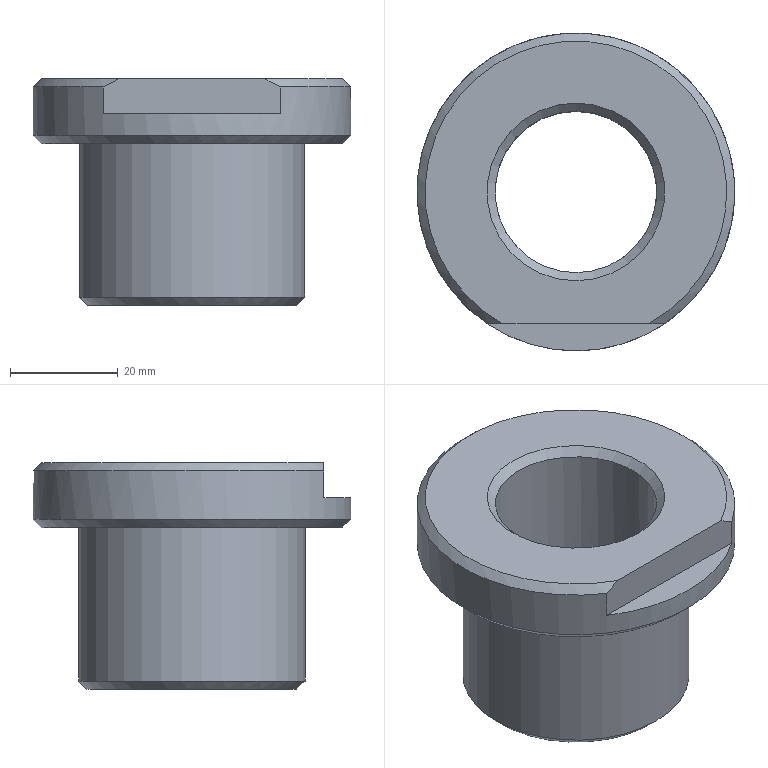Component | NX | BORING_SLEEVE | 1 solid | 13 faces | box 59 x 59 x 42 mm | volume 43221 mm3 | plane 5 | cone 5 | cylinder 3 | commonest cylinder face diameters 42 x1 59 x1 30 x1
STEP:
#1=CARTESIAN_POINT('',(0.,0.,0.));
#2=DIRECTION('',(0.,0.,1.));
#3=DIRECTION('',(1.,0.,0.));
#4=AXIS2_PLACEMENT_3D('',#1,#2,#3);
#5=CARTESIAN_POINT('',(34.,160.533,50.));
#6=VERTEX_POINT('',#5);
#7=CARTESIAN_POINT('',(34.,144.033,50.));
#8=DIRECTION('',(0.,0.,1.));
#9=DIRECTION('',(0.,1.,0.));
#10=AXIS2_PLACEMENT_3D('',#7,#8,#9);
#11=CIRCLE('',#10,16.5);
#12=CARTESIAN_POINT('',(34.,144.033,50.));
#13=DIRECTION('',(0.,0.,-1.));
#14=DIRECTION('',(0.,1.,0.));
#15=AXIS2_PLACEMENT_3D('',#12,#13,#14);
#16=PLANE('',#15);
#17=CARTESIAN_POINT('',(16.5,0.));
#18=CARTESIAN_POINT('',(16.5,-28.579));
#19=CARTESIAN_POINT('',(-8.25,-14.289));
#20=CARTESIAN_POINT('',(-33.,-0.));
#21=CARTESIAN_POINT('',(-8.25,14.289));
#22=CARTESIAN_POINT('',(16.5,28.579));
#23=CARTESIAN_POINT('',(16.5,0.));
#24=(BOUNDED_CURVE()B_SPLINE_CURVE(2,(#17,#18,#19,#20,#21,#22,#23),.UNSPECIFIED.,.T.,.F.)B_SPLINE_CURVE_WITH_KNOTS((1,2,2,2,2,1),(-2.094,0.,2.094,4.189,6.283,8.378),.UNSPECIFIED.)CURVE()GEOMETRIC_REPRESENTATION_ITEM()RATIONAL_B_SPLINE_CURVE((1.,0.5,1.,0.5,1.,0.5,1.))REPRESENTATION_ITEM(''));
#25=(GEOMETRIC_REPRESENTATION_CONTEXT(2)PARAMETRIC_REPRESENTATION_CONTEXT()REPRESENTATION_CONTEXT('',''));
#26=DEFINITIONAL_REPRESENTATION('',(#24),#25);
#27=PCURVE('',#16,#26);
#28=CARTESIAN_POINT('',(34.,144.033,51.5));
#29=DIRECTION('',(0.,0.,-1.));
#30=DIRECTION('',(0.,1.,0.));
#31=AXIS2_PLACEMENT_3D('',#28,#29,#30);
#32=CONICAL_SURFACE('',#31,15.,0.7854);
#33=CARTESIAN_POINT('',(6.283,1.5));
#34=DIRECTION('',(-1.,0.));
#35=VECTOR('',#34,1.);
#36=LINE('',#33,#35);
#37=(GEOMETRIC_REPRESENTATION_CONTEXT(2)PARAMETRIC_REPRESENTATION_CONTEXT()REPRESENTATION_CONTEXT('',''));
#38=DEFINITIONAL_REPRESENTATION('',(#36),#37);
#39=PCURVE('',#32,#38);
#40=SURFACE_CURVE('',#11,(#27,#39),.PCURVE_S1.);
#41=EDGE_CURVE('',#6,#6,#40,.T.);
#42=ORIENTED_EDGE('',*,*,#41,.T.);
#43=EDGE_LOOP('',(#42));
#44=FACE_BOUND('',#43,.T.);
#45=CARTESIAN_POINT('',(34.,163.533,50.));
#46=VERTEX_POINT('',#45);
#47=CARTESIAN_POINT('',(34.,144.033,50.));
#48=DIRECTION('',(0.,0.,-1.));
#49=DIRECTION('',(0.,1.,0.));
#50=AXIS2_PLACEMENT_3D('',#47,#48,#49);
#51=CIRCLE('',#50,19.5);
#52=CARTESIAN_POINT('',(0.,0.));
#53=DIRECTION('',(1.,0.));
#54=AXIS2_PLACEMENT_2D('',#52,#53);
#55=CIRCLE('',#54,19.5);
#56=(GEOMETRIC_REPRESENTATION_CONTEXT(2)PARAMETRIC_REPRESENTATION_CONTEXT()REPRESENTATION_CONTEXT('',''));
#57=DEFINITIONAL_REPRESENTATION('',(#55),#56);
#58=PCURVE('',#16,#57);
#59=CARTESIAN_POINT('',(34.,144.033,51.5));
#60=DIRECTION('',(0.,0.,1.));
#61=DIRECTION('',(0.,-1.,0.));
#62=AXIS2_PLACEMENT_3D('',#59,#60,#61);
#63=CONICAL_SURFACE('',#62,21.,0.7854);
#64=CARTESIAN_POINT('',(9.425,-1.5));
#65=DIRECTION('',(-1.,0.));
#66=VECTOR('',#65,1.);
#67=LINE('',#64,#66);
#68=(GEOMETRIC_REPRESENTATION_CONTEXT(2)PARAMETRIC_REPRESENTATION_CONTEXT()REPRESENTATION_CONTEXT('',''));
#69=DEFINITIONAL_REPRESENTATION('',(#67),#68);
#70=PCURVE('',#63,#69);
#71=SURFACE_CURVE('',#51,(#58,#70),.PCURVE_S1.);
#72=EDGE_CURVE('',#46,#46,#71,.T.);
#73=ORIENTED_EDGE('',*,*,#72,.T.);
#74=EDGE_LOOP('',(#73));
#75=FACE_BOUND('',#74,.T.);
#76=ADVANCED_FACE('',(#44,#75),#16,.T.);
#77=CARTESIAN_POINT('',(34.,165.033,51.5));
#78=VERTEX_POINT('',#77);
#79=CARTESIAN_POINT('',(34.,144.033,51.5));
#80=DIRECTION('',(0.,0.,1.));
#81=DIRECTION('',(0.,1.,0.));
#82=AXIS2_PLACEMENT_3D('',#79,#80,#81);
#83=CIRCLE('',#82,21.);
#84=CARTESIAN_POINT('',(34.,144.033,50.));
#85=DIRECTION('',(0.,0.,1.));
#86=DIRECTION('',(0.,-1.,0.));
#87=AXIS2_PLACEMENT_3D('',#84,#85,#86);
#88=CYLINDRICAL_SURFACE('',#87,21.);
#89=CARTESIAN_POINT('',(3.142,1.5));
#90=DIRECTION('',(1.,0.));
#91=VECTOR('',#90,1.);
#92=LINE('',#89,#91);
#93=(GEOMETRIC_REPRESENTATION_CONTEXT(2)PARAMETRIC_REPRESENTATION_CONTEXT()REPRESENTATION_CONTEXT('',''));
#94=DEFINITIONAL_REPRESENTATION('',(#92),#93);
#95=PCURVE('',#88,#94);
#96=CARTESIAN_POINT('',(3.142,0.));
#97=DIRECTION('',(1.,0.));
#98=VECTOR('',#97,1.);
#99=LINE('',#96,#98);
#100=(GEOMETRIC_REPRESENTATION_CONTEXT(2)PARAMETRIC_REPRESENTATION_CONTEXT()REPRESENTATION_CONTEXT('',''));
#101=DEFINITIONAL_REPRESENTATION('',(#99),#100);
#102=PCURVE('',#63,#101);
#103=SURFACE_CURVE('',#83,(#95,#102),.PCURVE_S1.);
#104=EDGE_CURVE('',#78,#78,#103,.T.);
#105=ORIENTED_EDGE('',*,*,#104,.T.);
#106=CARTESIAN_POINT('',(34.,165.033,80.));
#107=VERTEX_POINT('',#106);
#108=CARTESIAN_POINT('',(34.,165.033,51.5));
#109=CARTESIAN_POINT('',(34.,165.033,80.));
#110=B_SPLINE_CURVE_WITH_KNOTS('',1,(#108,#109),.UNSPECIFIED.,.F.,.F.,(2,2),(1.5,30.),.PIECEWISE_BEZIER_KNOTS.);
#111=CARTESIAN_POINT('',(9.425,0.));
#112=DIRECTION('',(0.,1.));
#113=VECTOR('',#112,1.);
#114=LINE('',#111,#113);
#115=(GEOMETRIC_REPRESENTATION_CONTEXT(2)PARAMETRIC_REPRESENTATION_CONTEXT()REPRESENTATION_CONTEXT('',''));
#116=DEFINITIONAL_REPRESENTATION('',(#114),#115);
#117=PCURVE('',#88,#116);
#118=CARTESIAN_POINT('',(3.142,0.));
#119=DIRECTION('',(0.,1.));
#120=VECTOR('',#119,1.);
#121=LINE('',#118,#120);
#122=(GEOMETRIC_REPRESENTATION_CONTEXT(2)PARAMETRIC_REPRESENTATION_CONTEXT()REPRESENTATION_CONTEXT('',''));
#123=DEFINITIONAL_REPRESENTATION('',(#121),#122);
#124=PCURVE('',#88,#123);
#125=SEAM_CURVE('',#110,(#117,#124),.PCURVE_S1.);
#126=EDGE_CURVE('',#78,#107,#125,.T.);
#127=ORIENTED_EDGE('',*,*,#126,.T.);
#128=CARTESIAN_POINT('',(34.,144.033,80.));
#129=DIRECTION('',(0.,0.,1.));
#130=DIRECTION('',(0.,1.,0.));
#131=AXIS2_PLACEMENT_3D('',#128,#129,#130);
#132=CIRCLE('',#131,21.);
#133=CARTESIAN_POINT('',(3.142,30.));
#134=DIRECTION('',(1.,0.));
#135=VECTOR('',#134,1.);
#136=LINE('',#133,#135);
#137=(GEOMETRIC_REPRESENTATION_CONTEXT(2)PARAMETRIC_REPRESENTATION_CONTEXT()REPRESENTATION_CONTEXT('',''));
#138=DEFINITIONAL_REPRESENTATION('',(#136),#137);
#139=PCURVE('',#88,#138);
#140=CARTESIAN_POINT('',(34.,144.033,80.));
#141=DIRECTION('',(0.,0.,-1.));
#142=DIRECTION('',(0.,1.,0.));
#143=AXIS2_PLACEMENT_3D('',#140,#141,#142);
#144=PLANE('',#143);
#145=CARTESIAN_POINT('',(21.,0.));
#146=CARTESIAN_POINT('',(21.,-36.373));
#147=CARTESIAN_POINT('',(-10.5,-18.187));
#148=CARTESIAN_POINT('',(-42.,-0.));
#149=CARTESIAN_POINT('',(-10.5,18.187));
#150=CARTESIAN_POINT('',(21.,36.373));
#151=CARTESIAN_POINT('',(21.,0.));
#152=(BOUNDED_CURVE()B_SPLINE_CURVE(2,(#145,#146,#147,#148,#149,#150,#151),.UNSPECIFIED.,.T.,.F.)B_SPLINE_CURVE_WITH_KNOTS((1,2,2,2,2,1),(-2.094,0.,2.094,4.189,6.283,8.378),.UNSPECIFIED.)CURVE()GEOMETRIC_REPRESENTATION_ITEM()RATIONAL_B_SPLINE_CURVE((1.,0.5,1.,0.5,1.,0.5,1.))REPRESENTATION_ITEM(''));
#153=(GEOMETRIC_REPRESENTATION_CONTEXT(2)PARAMETRIC_REPRESENTATION_CONTEXT()REPRESENTATION_CONTEXT('',''));
#154=DEFINITIONAL_REPRESENTATION('',(#152),#153);
#155=PCURVE('',#144,#154);
#156=SURFACE_CURVE('',#132,(#139,#155),.PCURVE_S1.);
#157=EDGE_CURVE('',#107,#107,#156,.T.);
#158=ORIENTED_EDGE('',*,*,#157,.F.);
#159=ORIENTED_EDGE('',*,*,#126,.F.);
#160=EDGE_LOOP('',(#105,#127,#158,#159));
#161=FACE_BOUND('',#160,.T.);
#162=ADVANCED_FACE('',(#161),#88,.T.);
#163=CARTESIAN_POINT('',(34.,127.533,92.));
#164=VERTEX_POINT('',#163);
#165=CARTESIAN_POINT('',(34.,144.033,92.));
#166=DIRECTION('',(0.,0.,-1.));
#167=DIRECTION('',(0.,-1.,0.));
#168=AXIS2_PLACEMENT_3D('',#165,#166,#167);
#169=CIRCLE('',#168,16.5);
#170=CARTESIAN_POINT('',(34.,144.033,92.));
#171=DIRECTION('',(0.,0.,1.));
#172=DIRECTION('',(0.,-1.,0.));
#173=AXIS2_PLACEMENT_3D('',#170,#171,#172);
#174=PLANE('',#173);
#175=CARTESIAN_POINT('',(16.5,0.));
#176=CARTESIAN_POINT('',(16.5,-28.579));
#177=CARTESIAN_POINT('',(-8.25,-14.289));
#178=CARTESIAN_POINT('',(-33.,-0.));
#179=CARTESIAN_POINT('',(-8.25,14.289));
#180=CARTESIAN_POINT('',(16.5,28.579));
#181=CARTESIAN_POINT('',(16.5,0.));
#182=(BOUNDED_CURVE()B_SPLINE_CURVE(2,(#175,#176,#177,#178,#179,#180,#181),.UNSPECIFIED.,.T.,.F.)B_SPLINE_CURVE_WITH_KNOTS((1,2,2,2,2,1),(-2.094,0.,2.094,4.189,6.283,8.378),.UNSPECIFIED.)CURVE()GEOMETRIC_REPRESENTATION_ITEM()RATIONAL_B_SPLINE_CURVE((1.,0.5,1.,0.5,1.,0.5,1.))REPRESENTATION_ITEM(''));
#183=(GEOMETRIC_REPRESENTATION_CONTEXT(2)PARAMETRIC_REPRESENTATION_CONTEXT()REPRESENTATION_CONTEXT('',''));
#184=DEFINITIONAL_REPRESENTATION('',(#182),#183);
#185=PCURVE('',#174,#184);
#186=CARTESIAN_POINT('',(34.,144.033,92.));
#187=DIRECTION('',(0.,0.,1.));
#188=DIRECTION('',(0.,-1.,0.));
#189=AXIS2_PLACEMENT_3D('',#186,#187,#188);
#190=CONICAL_SURFACE('',#189,16.5,0.7854);
#191=CARTESIAN_POINT('',(6.283,0.));
#192=DIRECTION('',(-1.,0.));
#193=VECTOR('',#192,1.);
#194=LINE('',#191,#193);
#195=(GEOMETRIC_REPRESENTATION_CONTEXT(2)PARAMETRIC_REPRESENTATION_CONTEXT()REPRESENTATION_CONTEXT('',''));
#196=DEFINITIONAL_REPRESENTATION('',(#194),#195);
#197=PCURVE('',#190,#196);
#198=SURFACE_CURVE('',#169,(#185,#197),.PCURVE_S1.);
#199=EDGE_CURVE('',#164,#164,#198,.T.);
#200=ORIENTED_EDGE('',*,*,#199,.T.);
#201=EDGE_LOOP('',(#200));
#202=FACE_BOUND('',#201,.T.);
#203=CARTESIAN_POINT('',(47.555,119.533,92.));
#204=VERTEX_POINT('',#203);
#205=CARTESIAN_POINT('',(20.445,119.533,92.));
#206=VERTEX_POINT('',#205);
#207=CARTESIAN_POINT('',(67.,119.533,92.));
#208=DIRECTION('',(-1.,-0.,0.));
#209=VECTOR('',#208,1.);
#210=LINE('',#207,#209);
#211=CARTESIAN_POINT('',(24.5,33.));
#212=DIRECTION('',(0.,-1.));
#213=VECTOR('',#212,1.);
#214=LINE('',#211,#213);
#215=(GEOMETRIC_REPRESENTATION_CONTEXT(2)PARAMETRIC_REPRESENTATION_CONTEXT()REPRESENTATION_CONTEXT('',''));
#216=DEFINITIONAL_REPRESENTATION('',(#214),#215);
#217=PCURVE('',#174,#216);
#218=CARTESIAN_POINT('',(67.,119.533,85.5));
#219=DIRECTION('',(-0.,1.,0.));
#220=DIRECTION('',(-1.,-0.,0.));
#221=AXIS2_PLACEMENT_3D('',#218,#219,#220);
#222=PLANE('',#221);
#223=CARTESIAN_POINT('',(0.,6.5));
#224=DIRECTION('',(1.,0.));
#225=VECTOR('',#224,1.);
#226=LINE('',#223,#225);
#227=(GEOMETRIC_REPRESENTATION_CONTEXT(2)PARAMETRIC_REPRESENTATION_CONTEXT()REPRESENTATION_CONTEXT('',''));
#228=DEFINITIONAL_REPRESENTATION('',(#226),#227);
#229=PCURVE('',#222,#228);
#230=SURFACE_CURVE('',#210,(#217,#229),.PCURVE_S1.);
#231=EDGE_CURVE('',#204,#206,#230,.T.);
#232=ORIENTED_EDGE('',*,*,#231,.F.);
#233=CARTESIAN_POINT('',(34.,144.033,92.));
#234=DIRECTION('',(0.,0.,1.));
#235=DIRECTION('',(0.,-1.,0.));
#236=AXIS2_PLACEMENT_3D('',#233,#234,#235);
#237=CIRCLE('',#236,28.);
#238=CARTESIAN_POINT('',(0.,0.));
#239=DIRECTION('',(1.,0.));
#240=AXIS2_PLACEMENT_2D('',#238,#239);
#241=CIRCLE('',#240,28.);
#242=(GEOMETRIC_REPRESENTATION_CONTEXT(2)PARAMETRIC_REPRESENTATION_CONTEXT()REPRESENTATION_CONTEXT('',''));
#243=DEFINITIONAL_REPRESENTATION('',(#241),#242);
#244=PCURVE('',#174,#243);
#245=CARTESIAN_POINT('',(34.,144.033,90.5));
#246=DIRECTION('',(0.,0.,-1.));
#247=DIRECTION('',(0.,1.,0.));
#248=AXIS2_PLACEMENT_3D('',#245,#246,#247);
#249=CONICAL_SURFACE('',#248,29.5,0.7854);
#250=CARTESIAN_POINT('',(9.425,-1.5));
#251=DIRECTION('',(-1.,-0.));
#252=VECTOR('',#251,1.);
#253=LINE('',#250,#252);
#254=(GEOMETRIC_REPRESENTATION_CONTEXT(2)PARAMETRIC_REPRESENTATION_CONTEXT()REPRESENTATION_CONTEXT('',''));
#255=DEFINITIONAL_REPRESENTATION('',(#253),#254);
#256=PCURVE('',#249,#255);
#257=SURFACE_CURVE('',#237,(#244,#256),.PCURVE_S1.);
#258=EDGE_CURVE('',#204,#206,#257,.T.);
#259=ORIENTED_EDGE('',*,*,#258,.T.);
#260=EDGE_LOOP('',(#232,#259));
#261=FACE_BOUND('',#260,.T.);
#262=ADVANCED_FACE('',(#202,#261),#174,.T.);
#263=CARTESIAN_POINT('',(34.,172.033,80.));
#264=VERTEX_POINT('',#263);
#265=CARTESIAN_POINT('',(34.,144.033,80.));
#266=DIRECTION('',(0.,0.,-1.));
#267=DIRECTION('',(0.,1.,0.));
#268=AXIS2_PLACEMENT_3D('',#265,#266,#267);
#269=CIRCLE('',#268,28.);
#270=CARTESIAN_POINT('',(0.,0.));
#271=DIRECTION('',(1.,0.));
#272=AXIS2_PLACEMENT_2D('',#270,#271);
#273=CIRCLE('',#272,28.);
#274=(GEOMETRIC_REPRESENTATION_CONTEXT(2)PARAMETRIC_REPRESENTATION_CONTEXT()REPRESENTATION_CONTEXT('',''));
#275=DEFINITIONAL_REPRESENTATION('',(#273),#274);
#276=PCURVE('',#144,#275);
#277=CARTESIAN_POINT('',(34.,144.033,81.5));
#278=DIRECTION('',(0.,0.,1.));
#279=DIRECTION('',(0.,-1.,0.));
#280=AXIS2_PLACEMENT_3D('',#277,#278,#279);
#281=CONICAL_SURFACE('',#280,29.5,0.7854);
#282=CARTESIAN_POINT('',(9.425,-1.5));
#283=DIRECTION('',(-1.,0.));
#284=VECTOR('',#283,1.);
#285=LINE('',#282,#284);
#286=(GEOMETRIC_REPRESENTATION_CONTEXT(2)PARAMETRIC_REPRESENTATION_CONTEXT()REPRESENTATION_CONTEXT('',''));
#287=DEFINITIONAL_REPRESENTATION('',(#285),#286);
#288=PCURVE('',#281,#287);
#289=SURFACE_CURVE('',#269,(#276,#288),.PCURVE_S1.);
#290=EDGE_CURVE('',#264,#264,#289,.T.);
#291=ORIENTED_EDGE('',*,*,#290,.T.);
#292=EDGE_LOOP('',(#291));
#293=FACE_BOUND('',#292,.T.);
#294=ORIENTED_EDGE('',*,*,#157,.T.);
#295=EDGE_LOOP('',(#294));
#296=FACE_BOUND('',#295,.T.);
#297=ADVANCED_FACE('',(#293,#296),#144,.T.);
#298=CARTESIAN_POINT('',(34.,173.533,81.5));
#299=VERTEX_POINT('',#298);
#300=CARTESIAN_POINT('',(17.568,119.533,81.5));
#301=VERTEX_POINT('',#300);
#302=CARTESIAN_POINT('',(34.,144.033,81.5));
#303=DIRECTION('',(0.,0.,1.));
#304=DIRECTION('',(0.,1.,0.));
#305=AXIS2_PLACEMENT_3D('',#302,#303,#304);
#306=CIRCLE('',#305,29.5);
#307=CARTESIAN_POINT('',(34.,144.033,80.));
#308=DIRECTION('',(0.,0.,1.));
#309=DIRECTION('',(0.,-1.,0.));
#310=AXIS2_PLACEMENT_3D('',#307,#308,#309);
#311=CYLINDRICAL_SURFACE('',#310,29.5);
#312=CARTESIAN_POINT('',(9.425,1.5));
#313=DIRECTION('',(1.,0.));
#314=VECTOR('',#313,1.);
#315=LINE('',#312,#314);
#316=(GEOMETRIC_REPRESENTATION_CONTEXT(2)PARAMETRIC_REPRESENTATION_CONTEXT()REPRESENTATION_CONTEXT('',''));
#317=DEFINITIONAL_REPRESENTATION('',(#315),#316);
#318=PCURVE('',#311,#317);
#319=CARTESIAN_POINT('',(3.142,0.));
#320=DIRECTION('',(1.,0.));
#321=VECTOR('',#320,1.);
#322=LINE('',#319,#321);
#323=(GEOMETRIC_REPRESENTATION_CONTEXT(2)PARAMETRIC_REPRESENTATION_CONTEXT()REPRESENTATION_CONTEXT('',''));
#324=DEFINITIONAL_REPRESENTATION('',(#322),#323);
#325=PCURVE('',#281,#324);
#326=SURFACE_CURVE('',#306,(#318,#325),.PCURVE_S1.);
#327=EDGE_CURVE('',#299,#301,#326,.T.);
#328=ORIENTED_EDGE('',*,*,#327,.T.);
#329=CARTESIAN_POINT('',(17.568,119.533,85.5));
#330=VERTEX_POINT('',#329);
#331=CARTESIAN_POINT('',(17.568,119.533,81.5));
#332=CARTESIAN_POINT('',(17.568,119.533,85.5));
#333=B_SPLINE_CURVE_WITH_KNOTS('',1,(#331,#332),.UNSPECIFIED.,.F.,.F.,(2,2),(1.5,5.5),.PIECEWISE_BEZIER_KNOTS.);
#334=CARTESIAN_POINT('',(11.976,0.));
#335=DIRECTION('',(0.,1.));
#336=VECTOR('',#335,1.);
#337=LINE('',#334,#336);
#338=(GEOMETRIC_REPRESENTATION_CONTEXT(2)PARAMETRIC_REPRESENTATION_CONTEXT()REPRESENTATION_CONTEXT('',''));
#339=DEFINITIONAL_REPRESENTATION('',(#337),#338);
#340=PCURVE('',#311,#339);
#341=CARTESIAN_POINT('',(5.692,0.));
#342=DIRECTION('',(0.,1.));
#343=VECTOR('',#342,1.);
#344=LINE('',#341,#343);
#345=(GEOMETRIC_REPRESENTATION_CONTEXT(2)PARAMETRIC_REPRESENTATION_CONTEXT()REPRESENTATION_CONTEXT('',''));
#346=DEFINITIONAL_REPRESENTATION('',(#344),#345);
#347=PCURVE('',#311,#346);
#348=SEAM_CURVE('',#333,(#340,#347),.PCURVE_S1.);
#349=EDGE_CURVE('',#301,#330,#348,.T.);
#350=ORIENTED_EDGE('',*,*,#349,.T.);
#351=CARTESIAN_POINT('',(17.568,119.533,90.5));
#352=VERTEX_POINT('',#351);
#353=CARTESIAN_POINT('',(17.568,119.533,80.));
#354=DIRECTION('',(0.,0.,-1.));
#355=VECTOR('',#354,1.);
#356=LINE('',#353,#355);
#357=CARTESIAN_POINT('',(11.976,0.));
#358=DIRECTION('',(0.,-1.));
#359=VECTOR('',#358,1.);
#360=LINE('',#357,#359);
#361=(GEOMETRIC_REPRESENTATION_CONTEXT(2)PARAMETRIC_REPRESENTATION_CONTEXT()REPRESENTATION_CONTEXT('',''));
#362=DEFINITIONAL_REPRESENTATION('',(#360),#361);
#363=PCURVE('',#311,#362);
#364=CARTESIAN_POINT('',(49.432,-5.5));
#365=DIRECTION('',(0.,-1.));
#366=VECTOR('',#365,1.);
#367=LINE('',#364,#366);
#368=(GEOMETRIC_REPRESENTATION_CONTEXT(2)PARAMETRIC_REPRESENTATION_CONTEXT()REPRESENTATION_CONTEXT('',''));
#369=DEFINITIONAL_REPRESENTATION('',(#367),#368);
#370=PCURVE('',#222,#369);
#371=SURFACE_CURVE('',#356,(#363,#370),.PCURVE_S1.);
#372=EDGE_CURVE('',#352,#330,#371,.T.);
#373=ORIENTED_EDGE('',*,*,#372,.F.);
#374=CARTESIAN_POINT('',(50.432,119.533,90.5));
#375=VERTEX_POINT('',#374);
#376=CARTESIAN_POINT('',(34.,144.033,90.5));
#377=DIRECTION('',(0.,0.,-1.));
#378=DIRECTION('',(0.,-1.,0.));
#379=AXIS2_PLACEMENT_3D('',#376,#377,#378);
#380=CIRCLE('',#379,29.5);
#381=CARTESIAN_POINT('',(12.566,10.5));
#382=DIRECTION('',(-1.,0.));
#383=VECTOR('',#382,1.);
#384=LINE('',#381,#383);
#385=(GEOMETRIC_REPRESENTATION_CONTEXT(2)PARAMETRIC_REPRESENTATION_CONTEXT()REPRESENTATION_CONTEXT('',''));
#386=DEFINITIONAL_REPRESENTATION('',(#384),#385);
#387=PCURVE('',#311,#386);
#388=CARTESIAN_POINT('',(3.142,0.));
#389=DIRECTION('',(1.,-0.));
#390=VECTOR('',#389,1.);
#391=LINE('',#388,#390);
#392=(GEOMETRIC_REPRESENTATION_CONTEXT(2)PARAMETRIC_REPRESENTATION_CONTEXT()REPRESENTATION_CONTEXT('',''));
#393=DEFINITIONAL_REPRESENTATION('',(#391),#392);
#394=PCURVE('',#249,#393);
#395=SURFACE_CURVE('',#380,(#387,#394),.PCURVE_S1.);
#396=EDGE_CURVE('',#352,#375,#395,.T.);
#397=ORIENTED_EDGE('',*,*,#396,.T.);
#398=CARTESIAN_POINT('',(50.432,119.533,85.5));
#399=VERTEX_POINT('',#398);
#400=CARTESIAN_POINT('',(50.432,119.533,80.));
#401=DIRECTION('',(0.,0.,1.));
#402=VECTOR('',#401,1.);
#403=LINE('',#400,#402);
#404=CARTESIAN_POINT('',(6.874,0.));
#405=DIRECTION('',(0.,1.));
#406=VECTOR('',#405,1.);
#407=LINE('',#404,#406);
#408=(GEOMETRIC_REPRESENTATION_CONTEXT(2)PARAMETRIC_REPRESENTATION_CONTEXT()REPRESENTATION_CONTEXT('',''));
#409=DEFINITIONAL_REPRESENTATION('',(#407),#408);
#410=PCURVE('',#311,#409);
#411=CARTESIAN_POINT('',(16.568,-5.5));
#412=DIRECTION('',(0.,1.));
#413=VECTOR('',#412,1.);
#414=LINE('',#411,#413);
#415=(GEOMETRIC_REPRESENTATION_CONTEXT(2)PARAMETRIC_REPRESENTATION_CONTEXT()REPRESENTATION_CONTEXT('',''));
#416=DEFINITIONAL_REPRESENTATION('',(#414),#415);
#417=PCURVE('',#222,#416);
#418=SURFACE_CURVE('',#403,(#410,#417),.PCURVE_S1.);
#419=EDGE_CURVE('',#399,#375,#418,.T.);
#420=ORIENTED_EDGE('',*,*,#419,.F.);
#421=CARTESIAN_POINT('',(34.,144.033,85.5));
#422=DIRECTION('',(0.,0.,-1.));
#423=DIRECTION('',(0.,-1.,0.));
#424=AXIS2_PLACEMENT_3D('',#421,#422,#423);
#425=CIRCLE('',#424,29.5);
#426=CARTESIAN_POINT('',(12.566,5.5));
#427=DIRECTION('',(-1.,0.));
#428=VECTOR('',#427,1.);
#429=LINE('',#426,#428);
#430=(GEOMETRIC_REPRESENTATION_CONTEXT(2)PARAMETRIC_REPRESENTATION_CONTEXT()REPRESENTATION_CONTEXT('',''));
#431=DEFINITIONAL_REPRESENTATION('',(#429),#430);
#432=PCURVE('',#311,#431);
#433=CARTESIAN_POINT('',(34.,144.033,85.5));
#434=DIRECTION('',(0.,0.,1.));
#435=DIRECTION('',(0.,-1.,0.));
#436=AXIS2_PLACEMENT_3D('',#433,#434,#435);
#437=PLANE('',#436);
#438=CARTESIAN_POINT('',(29.5,0.));
#439=CARTESIAN_POINT('',(29.5,-51.095));
#440=CARTESIAN_POINT('',(-14.75,-25.548));
#441=CARTESIAN_POINT('',(-59.,-0.));
#442=CARTESIAN_POINT('',(-14.75,25.548));
#443=CARTESIAN_POINT('',(29.5,51.095));
#444=CARTESIAN_POINT('',(29.5,0.));
#445=(BOUNDED_CURVE()B_SPLINE_CURVE(2,(#438,#439,#440,#441,#442,#443,#444),.UNSPECIFIED.,.T.,.F.)B_SPLINE_CURVE_WITH_KNOTS((1,2,2,2,2,1),(-2.094,0.,2.094,4.189,6.283,8.378),.UNSPECIFIED.)CURVE()GEOMETRIC_REPRESENTATION_ITEM()RATIONAL_B_SPLINE_CURVE((1.,0.5,1.,0.5,1.,0.5,1.))REPRESENTATION_ITEM(''));
#446=(GEOMETRIC_REPRESENTATION_CONTEXT(2)PARAMETRIC_REPRESENTATION_CONTEXT()REPRESENTATION_CONTEXT('',''));
#447=DEFINITIONAL_REPRESENTATION('',(#445),#446);
#448=PCURVE('',#437,#447);
#449=SURFACE_CURVE('',#425,(#432,#448),.PCURVE_S1.);
#450=EDGE_CURVE('',#399,#330,#449,.T.);
#451=ORIENTED_EDGE('',*,*,#450,.T.);
#452=ORIENTED_EDGE('',*,*,#349,.F.);
#453=CARTESIAN_POINT('',(34.,144.033,81.5));
#454=DIRECTION('',(0.,0.,1.));
#455=DIRECTION('',(0.,1.,0.));
#456=AXIS2_PLACEMENT_3D('',#453,#454,#455);
#457=CIRCLE('',#456,29.5);
#458=CARTESIAN_POINT('',(3.142,1.5));
#459=DIRECTION('',(1.,0.));
#460=VECTOR('',#459,1.);
#461=LINE('',#458,#460);
#462=(GEOMETRIC_REPRESENTATION_CONTEXT(2)PARAMETRIC_REPRESENTATION_CONTEXT()REPRESENTATION_CONTEXT('',''));
#463=DEFINITIONAL_REPRESENTATION('',(#461),#462);
#464=PCURVE('',#311,#463);
#465=CARTESIAN_POINT('',(3.142,0.));
#466=DIRECTION('',(1.,0.));
#467=VECTOR('',#466,1.);
#468=LINE('',#465,#467);
#469=(GEOMETRIC_REPRESENTATION_CONTEXT(2)PARAMETRIC_REPRESENTATION_CONTEXT()REPRESENTATION_CONTEXT('',''));
#470=DEFINITIONAL_REPRESENTATION('',(#468),#469);
#471=PCURVE('',#281,#470);
#472=SURFACE_CURVE('',#457,(#464,#471),.PCURVE_S1.);
#473=EDGE_CURVE('',#301,#299,#472,.T.);
#474=ORIENTED_EDGE('',*,*,#473,.T.);
#475=EDGE_LOOP('',(#328,#350,#373,#397,#420,#451,#452,#474));
#476=FACE_BOUND('',#475,.T.);
#477=ADVANCED_FACE('',(#476),#311,.T.);
#478=CARTESIAN_POINT('',(34.,159.033,51.5));
#479=VERTEX_POINT('',#478);
#480=CARTESIAN_POINT('',(34.,144.033,51.5));
#481=DIRECTION('',(0.,0.,-1.));
#482=DIRECTION('',(0.,1.,0.));
#483=AXIS2_PLACEMENT_3D('',#480,#481,#482);
#484=CIRCLE('',#483,15.);
#485=CARTESIAN_POINT('',(34.,144.033,92.));
#486=DIRECTION('',(0.,0.,-1.));
#487=DIRECTION('',(0.,1.,0.));
#488=AXIS2_PLACEMENT_3D('',#485,#486,#487);
#489=CYLINDRICAL_SURFACE('',#488,15.);
#490=CARTESIAN_POINT('',(0.,40.5));
#491=DIRECTION('',(1.,0.));
#492=VECTOR('',#491,1.);
#493=LINE('',#490,#492);
#494=(GEOMETRIC_REPRESENTATION_CONTEXT(2)PARAMETRIC_REPRESENTATION_CONTEXT()REPRESENTATION_CONTEXT('',''));
#495=DEFINITIONAL_REPRESENTATION('',(#493),#494);
#496=PCURVE('',#489,#495);
#497=CARTESIAN_POINT('',(0.,0.));
#498=DIRECTION('',(1.,0.));
#499=VECTOR('',#498,1.);
#500=LINE('',#497,#499);
#501=(GEOMETRIC_REPRESENTATION_CONTEXT(2)PARAMETRIC_REPRESENTATION_CONTEXT()REPRESENTATION_CONTEXT('',''));
#502=DEFINITIONAL_REPRESENTATION('',(#500),#501);
#503=PCURVE('',#32,#502);
#504=SURFACE_CURVE('',#484,(#496,#503),.PCURVE_S1.);
#505=EDGE_CURVE('',#479,#479,#504,.T.);
#506=ORIENTED_EDGE('',*,*,#505,.F.);
#507=CARTESIAN_POINT('',(34.,159.033,90.5));
#508=VERTEX_POINT('',#507);
#509=CARTESIAN_POINT('',(34.,159.033,90.5));
#510=CARTESIAN_POINT('',(34.,159.033,51.5));
#511=B_SPLINE_CURVE_WITH_KNOTS('',1,(#509,#510),.UNSPECIFIED.,.F.,.F.,(2,2),(1.5,40.5),.PIECEWISE_BEZIER_KNOTS.);
#512=CARTESIAN_POINT('',(0.,0.));
#513=DIRECTION('',(0.,1.));
#514=VECTOR('',#513,1.);
#515=LINE('',#512,#514);
#516=(GEOMETRIC_REPRESENTATION_CONTEXT(2)PARAMETRIC_REPRESENTATION_CONTEXT()REPRESENTATION_CONTEXT('',''));
#517=DEFINITIONAL_REPRESENTATION('',(#515),#516);
#518=PCURVE('',#489,#517);
#519=CARTESIAN_POINT('',(6.283,0.));
#520=DIRECTION('',(0.,1.));
#521=VECTOR('',#520,1.);
#522=LINE('',#519,#521);
#523=(GEOMETRIC_REPRESENTATION_CONTEXT(2)PARAMETRIC_REPRESENTATION_CONTEXT()REPRESENTATION_CONTEXT('',''));
#524=DEFINITIONAL_REPRESENTATION('',(#522),#523);
#525=PCURVE('',#489,#524);
#526=SEAM_CURVE('',#511,(#518,#525),.PCURVE_S1.);
#527=EDGE_CURVE('',#508,#479,#526,.T.);
#528=ORIENTED_EDGE('',*,*,#527,.F.);
#529=CARTESIAN_POINT('',(34.,129.033,90.5));
#530=VERTEX_POINT('',#529);
#531=CARTESIAN_POINT('',(34.,144.033,90.5));
#532=DIRECTION('',(0.,0.,1.));
#533=DIRECTION('',(0.,-1.,0.));
#534=AXIS2_PLACEMENT_3D('',#531,#532,#533);
#535=CIRCLE('',#534,15.);
#536=CARTESIAN_POINT('',(3.142,1.5));
#537=DIRECTION('',(-1.,0.));
#538=VECTOR('',#537,1.);
#539=LINE('',#536,#538);
#540=(GEOMETRIC_REPRESENTATION_CONTEXT(2)PARAMETRIC_REPRESENTATION_CONTEXT()REPRESENTATION_CONTEXT('',''));
#541=DEFINITIONAL_REPRESENTATION('',(#539),#540);
#542=PCURVE('',#489,#541);
#543=CARTESIAN_POINT('',(0.,-1.5));
#544=DIRECTION('',(1.,0.));
#545=VECTOR('',#544,1.);
#546=LINE('',#543,#545);
#547=(GEOMETRIC_REPRESENTATION_CONTEXT(2)PARAMETRIC_REPRESENTATION_CONTEXT()REPRESENTATION_CONTEXT('',''));
#548=DEFINITIONAL_REPRESENTATION('',(#546),#547);
#549=PCURVE('',#190,#548);
#550=SURFACE_CURVE('',#535,(#542,#549),.PCURVE_S1.);
#551=EDGE_CURVE('',#530,#508,#550,.T.);
#552=ORIENTED_EDGE('',*,*,#551,.F.);
#553=CARTESIAN_POINT('',(34.,144.033,90.5));
#554=DIRECTION('',(0.,0.,1.));
#555=DIRECTION('',(0.,-1.,0.));
#556=AXIS2_PLACEMENT_3D('',#553,#554,#555);
#557=CIRCLE('',#556,15.);
#558=CARTESIAN_POINT('',(9.425,1.5));
#559=DIRECTION('',(-1.,0.));
#560=VECTOR('',#559,1.);
#561=LINE('',#558,#560);
#562=(GEOMETRIC_REPRESENTATION_CONTEXT(2)PARAMETRIC_REPRESENTATION_CONTEXT()REPRESENTATION_CONTEXT('',''));
#563=DEFINITIONAL_REPRESENTATION('',(#561),#562);
#564=PCURVE('',#489,#563);
#565=CARTESIAN_POINT('',(0.,-1.5));
#566=DIRECTION('',(1.,0.));
#567=VECTOR('',#566,1.);
#568=LINE('',#565,#567);
#569=(GEOMETRIC_REPRESENTATION_CONTEXT(2)PARAMETRIC_REPRESENTATION_CONTEXT()REPRESENTATION_CONTEXT('',''));
#570=DEFINITIONAL_REPRESENTATION('',(#568),#569);
#571=PCURVE('',#190,#570);
#572=SURFACE_CURVE('',#557,(#564,#571),.PCURVE_S1.);
#573=EDGE_CURVE('',#508,#530,#572,.T.);
#574=ORIENTED_EDGE('',*,*,#573,.F.);
#575=ORIENTED_EDGE('',*,*,#527,.T.);
#576=EDGE_LOOP('',(#506,#528,#552,#574,#575));
#577=FACE_BOUND('',#576,.F.);
#578=ADVANCED_FACE('',(#577),#489,.F.);
#579=ORIENTED_EDGE('',*,*,#419,.T.);
#580=CARTESIAN_POINT('',(50.432,119.533,90.5));
#581=CARTESIAN_POINT('',(49.487,119.533,91.026));
#582=CARTESIAN_POINT('',(48.529,119.533,91.529));
#583=CARTESIAN_POINT('',(47.555,119.533,92.));
#584=B_SPLINE_CURVE_WITH_KNOTS('',3,(#580,#581,#582,#583),.UNSPECIFIED.,.F.,.F.,(4,4),(0.,1.),.PIECEWISE_BEZIER_KNOTS.);
#585=CARTESIAN_POINT('',(16.568,5.));
#586=CARTESIAN_POINT('',(17.513,5.526));
#587=CARTESIAN_POINT('',(18.471,6.029));
#588=CARTESIAN_POINT('',(19.445,6.5));
#589=B_SPLINE_CURVE_WITH_KNOTS('',3,(#585,#586,#587,#588),.UNSPECIFIED.,.F.,.F.,(4,4),(0.,1.),.PIECEWISE_BEZIER_KNOTS.);
#590=(GEOMETRIC_REPRESENTATION_CONTEXT(2)PARAMETRIC_REPRESENTATION_CONTEXT()REPRESENTATION_CONTEXT('',''));
#591=DEFINITIONAL_REPRESENTATION('',(#589),#590);
#592=PCURVE('',#222,#591);
#593=CARTESIAN_POINT('',(8.834,-0.));
#594=CARTESIAN_POINT('',(8.919,-1.5));
#595=B_SPLINE_CURVE_WITH_KNOTS('',1,(#593,#594),.UNSPECIFIED.,.F.,.F.,(2,2),(0.,1.),.PIECEWISE_BEZIER_KNOTS.);
#596=(GEOMETRIC_REPRESENTATION_CONTEXT(2)PARAMETRIC_REPRESENTATION_CONTEXT()REPRESENTATION_CONTEXT('',''));
#597=DEFINITIONAL_REPRESENTATION('',(#595),#596);
#598=PCURVE('',#249,#597);
#599=SURFACE_CURVE('',#584,(#592,#598),.PCURVE_S1.);
#600=EDGE_CURVE('',#375,#204,#599,.T.);
#601=ORIENTED_EDGE('',*,*,#600,.T.);
#602=ORIENTED_EDGE('',*,*,#231,.T.);
#603=CARTESIAN_POINT('',(20.445,119.533,92.));
#604=CARTESIAN_POINT('',(19.471,119.533,91.529));
#605=CARTESIAN_POINT('',(18.513,119.533,91.026));
#606=CARTESIAN_POINT('',(17.568,119.533,90.5));
#607=B_SPLINE_CURVE_WITH_KNOTS('',3,(#603,#604,#605,#606),.UNSPECIFIED.,.F.,.F.,(4,4),(0.,1.),.PIECEWISE_BEZIER_KNOTS.);
#608=CARTESIAN_POINT('',(46.555,6.5));
#609=CARTESIAN_POINT('',(47.529,6.029));
#610=CARTESIAN_POINT('',(48.487,5.526));
#611=CARTESIAN_POINT('',(49.432,5.));
#612=B_SPLINE_CURVE_WITH_KNOTS('',3,(#608,#609,#610,#611),.UNSPECIFIED.,.F.,.F.,(4,4),(0.,1.),.PIECEWISE_BEZIER_KNOTS.);
#613=(GEOMETRIC_REPRESENTATION_CONTEXT(2)PARAMETRIC_REPRESENTATION_CONTEXT()REPRESENTATION_CONTEXT('',''));
#614=DEFINITIONAL_REPRESENTATION('',(#612),#613);
#615=PCURVE('',#222,#614);
#616=CARTESIAN_POINT('',(3.647,-1.5));
#617=CARTESIAN_POINT('',(3.732,-0.));
#618=B_SPLINE_CURVE_WITH_KNOTS('',1,(#616,#617),.UNSPECIFIED.,.F.,.F.,(2,2),(0.,1.),.PIECEWISE_BEZIER_KNOTS.);
#619=(GEOMETRIC_REPRESENTATION_CONTEXT(2)PARAMETRIC_REPRESENTATION_CONTEXT()REPRESENTATION_CONTEXT('',''));
#620=DEFINITIONAL_REPRESENTATION('',(#618),#619);
#621=PCURVE('',#249,#620);
#622=SURFACE_CURVE('',#607,(#615,#621),.PCURVE_S1.);
#623=EDGE_CURVE('',#206,#352,#622,.T.);
#624=ORIENTED_EDGE('',*,*,#623,.T.);
#625=ORIENTED_EDGE('',*,*,#372,.T.);
#626=CARTESIAN_POINT('',(67.,119.533,85.5));
#627=DIRECTION('',(1.,0.,0.));
#628=VECTOR('',#627,1.);
#629=LINE('',#626,#628);
#630=CARTESIAN_POINT('',(0.,0.));
#631=DIRECTION('',(-1.,0.));
#632=VECTOR('',#631,1.);
#633=LINE('',#630,#632);
#634=(GEOMETRIC_REPRESENTATION_CONTEXT(2)PARAMETRIC_REPRESENTATION_CONTEXT()REPRESENTATION_CONTEXT('',''));
#635=DEFINITIONAL_REPRESENTATION('',(#633),#634);
#636=PCURVE('',#222,#635);
#637=CARTESIAN_POINT('',(24.5,33.));
#638=DIRECTION('',(-0.,1.));
#639=VECTOR('',#638,1.);
#640=LINE('',#637,#639);
#641=(GEOMETRIC_REPRESENTATION_CONTEXT(2)PARAMETRIC_REPRESENTATION_CONTEXT()REPRESENTATION_CONTEXT('',''));
#642=DEFINITIONAL_REPRESENTATION('',(#640),#641);
#643=PCURVE('',#437,#642);
#644=SURFACE_CURVE('',#629,(#636,#643),.PCURVE_S1.);
#645=EDGE_CURVE('',#330,#399,#644,.T.);
#646=ORIENTED_EDGE('',*,*,#645,.T.);
#647=EDGE_LOOP('',(#579,#601,#602,#624,#625,#646));
#648=FACE_BOUND('',#647,.T.);
#649=ADVANCED_FACE('',(#648),#222,.F.);
#650=ORIENTED_EDGE('',*,*,#645,.F.);
#651=ORIENTED_EDGE('',*,*,#450,.F.);
#652=EDGE_LOOP('',(#650,#651));
#653=FACE_BOUND('',#652,.T.);
#654=ADVANCED_FACE('',(#653),#437,.T.);
#655=ORIENTED_EDGE('',*,*,#41,.T.);
#656=CARTESIAN_POINT('',(34.,159.033,51.5));
#657=CARTESIAN_POINT('',(34.,160.533,50.));
#658=B_SPLINE_CURVE_WITH_KNOTS('',1,(#656,#657),.UNSPECIFIED.,.F.,.F.,(2,2),(0.,2.121),.PIECEWISE_BEZIER_KNOTS.);
#659=CARTESIAN_POINT('',(0.,0.));
#660=DIRECTION('',(0.,1.));
#661=VECTOR('',#660,1.);
#662=LINE('',#659,#661);
#663=(GEOMETRIC_REPRESENTATION_CONTEXT(2)PARAMETRIC_REPRESENTATION_CONTEXT()REPRESENTATION_CONTEXT('',''));
#664=DEFINITIONAL_REPRESENTATION('',(#662),#663);
#665=PCURVE('',#32,#664);
#666=CARTESIAN_POINT('',(6.283,0.));
#667=DIRECTION('',(0.,1.));
#668=VECTOR('',#667,1.);
#669=LINE('',#666,#668);
#670=(GEOMETRIC_REPRESENTATION_CONTEXT(2)PARAMETRIC_REPRESENTATION_CONTEXT()REPRESENTATION_CONTEXT('',''));
#671=DEFINITIONAL_REPRESENTATION('',(#669),#670);
#672=PCURVE('',#32,#671);
#673=SEAM_CURVE('',#658,(#665,#672),.PCURVE_S1.);
#674=EDGE_CURVE('',#479,#6,#673,.T.);
#675=ORIENTED_EDGE('',*,*,#674,.F.);
#676=ORIENTED_EDGE('',*,*,#505,.T.);
#677=ORIENTED_EDGE('',*,*,#674,.T.);
#678=EDGE_LOOP('',(#655,#675,#676,#677));
#679=FACE_BOUND('',#678,.F.);
#680=ADVANCED_FACE('',(#679),#32,.F.);
#681=ORIENTED_EDGE('',*,*,#72,.F.);
#682=CARTESIAN_POINT('',(34.,163.533,50.));
#683=CARTESIAN_POINT('',(34.,165.033,51.5));
#684=B_SPLINE_CURVE_WITH_KNOTS('',1,(#682,#683),.UNSPECIFIED.,.F.,.F.,(2,2),(-2.121,0.),.PIECEWISE_BEZIER_KNOTS.);
#685=CARTESIAN_POINT('',(9.425,0.));
#686=DIRECTION('',(0.,1.));
#687=VECTOR('',#686,1.);
#688=LINE('',#685,#687);
#689=(GEOMETRIC_REPRESENTATION_CONTEXT(2)PARAMETRIC_REPRESENTATION_CONTEXT()REPRESENTATION_CONTEXT('',''));
#690=DEFINITIONAL_REPRESENTATION('',(#688),#689);
#691=PCURVE('',#63,#690);
#692=CARTESIAN_POINT('',(3.142,0.));
#693=DIRECTION('',(0.,1.));
#694=VECTOR('',#693,1.);
#695=LINE('',#692,#694);
#696=(GEOMETRIC_REPRESENTATION_CONTEXT(2)PARAMETRIC_REPRESENTATION_CONTEXT()REPRESENTATION_CONTEXT('',''));
#697=DEFINITIONAL_REPRESENTATION('',(#695),#696);
#698=PCURVE('',#63,#697);
#699=SEAM_CURVE('',#684,(#691,#698),.PCURVE_S1.);
#700=EDGE_CURVE('',#46,#78,#699,.T.);
#701=ORIENTED_EDGE('',*,*,#700,.T.);
#702=ORIENTED_EDGE('',*,*,#104,.F.);
#703=ORIENTED_EDGE('',*,*,#700,.F.);
#704=EDGE_LOOP('',(#681,#701,#702,#703));
#705=FACE_BOUND('',#704,.T.);
#706=ADVANCED_FACE('',(#705),#63,.T.);
#707=ORIENTED_EDGE('',*,*,#290,.F.);
#708=CARTESIAN_POINT('',(34.,172.033,80.));
#709=CARTESIAN_POINT('',(34.,173.533,81.5));
#710=B_SPLINE_CURVE_WITH_KNOTS('',1,(#708,#709),.UNSPECIFIED.,.F.,.F.,(2,2),(-2.121,0.),.PIECEWISE_BEZIER_KNOTS.);
#711=CARTESIAN_POINT('',(9.425,0.));
#712=DIRECTION('',(0.,1.));
#713=VECTOR('',#712,1.);
#714=LINE('',#711,#713);
#715=(GEOMETRIC_REPRESENTATION_CONTEXT(2)PARAMETRIC_REPRESENTATION_CONTEXT()REPRESENTATION_CONTEXT('',''));
#716=DEFINITIONAL_REPRESENTATION('',(#714),#715);
#717=PCURVE('',#281,#716);
#718=CARTESIAN_POINT('',(3.142,0.));
#719=DIRECTION('',(0.,1.));
#720=VECTOR('',#719,1.);
#721=LINE('',#718,#720);
#722=(GEOMETRIC_REPRESENTATION_CONTEXT(2)PARAMETRIC_REPRESENTATION_CONTEXT()REPRESENTATION_CONTEXT('',''));
#723=DEFINITIONAL_REPRESENTATION('',(#721),#722);
#724=PCURVE('',#281,#723);
#725=SEAM_CURVE('',#710,(#717,#724),.PCURVE_S1.);
#726=EDGE_CURVE('',#264,#299,#725,.T.);
#727=ORIENTED_EDGE('',*,*,#726,.T.);
#728=ORIENTED_EDGE('',*,*,#473,.F.);
#729=ORIENTED_EDGE('',*,*,#327,.F.);
#730=ORIENTED_EDGE('',*,*,#726,.F.);
#731=EDGE_LOOP('',(#707,#727,#728,#729,#730));
#732=FACE_BOUND('',#731,.T.);
#733=ADVANCED_FACE('',(#732),#281,.T.);
#734=ORIENTED_EDGE('',*,*,#573,.T.);
#735=CARTESIAN_POINT('',(34.,129.033,90.5));
#736=CARTESIAN_POINT('',(34.,127.533,92.));
#737=B_SPLINE_CURVE_WITH_KNOTS('',1,(#735,#736),.UNSPECIFIED.,.F.,.F.,(2,2),(-2.121,0.),.PIECEWISE_BEZIER_KNOTS.);
#738=CARTESIAN_POINT('',(6.283,0.));
#739=DIRECTION('',(0.,1.));
#740=VECTOR('',#739,1.);
#741=LINE('',#738,#740);
#742=(GEOMETRIC_REPRESENTATION_CONTEXT(2)PARAMETRIC_REPRESENTATION_CONTEXT()REPRESENTATION_CONTEXT('',''));
#743=DEFINITIONAL_REPRESENTATION('',(#741),#742);
#744=PCURVE('',#190,#743);
#745=CARTESIAN_POINT('',(0.,0.));
#746=DIRECTION('',(0.,1.));
#747=VECTOR('',#746,1.);
#748=LINE('',#745,#747);
#749=(GEOMETRIC_REPRESENTATION_CONTEXT(2)PARAMETRIC_REPRESENTATION_CONTEXT()REPRESENTATION_CONTEXT('',''));
#750=DEFINITIONAL_REPRESENTATION('',(#748),#749);
#751=PCURVE('',#190,#750);
#752=SEAM_CURVE('',#737,(#744,#751),.PCURVE_S1.);
#753=EDGE_CURVE('',#530,#164,#752,.T.);
#754=ORIENTED_EDGE('',*,*,#753,.T.);
#755=ORIENTED_EDGE('',*,*,#199,.T.);
#756=ORIENTED_EDGE('',*,*,#753,.F.);
#757=ORIENTED_EDGE('',*,*,#551,.T.);
#758=EDGE_LOOP('',(#734,#754,#755,#756,#757));
#759=FACE_BOUND('',#758,.F.);
#760=ADVANCED_FACE('',(#759),#190,.F.);
#761=ORIENTED_EDGE('',*,*,#623,.F.);
#762=ORIENTED_EDGE('',*,*,#258,.F.);
#763=ORIENTED_EDGE('',*,*,#600,.F.);
#764=ORIENTED_EDGE('',*,*,#396,.F.);
#765=EDGE_LOOP('',(#761,#762,#763,#764));
#766=FACE_BOUND('',#765,.T.);
#767=ADVANCED_FACE('',(#766),#249,.T.);
#768=CLOSED_SHELL('',(#76,#162,#262,#297,#477,#578,#649,#654,#680,#706,#733,#760,#767));
#769=MANIFOLD_SOLID_BREP('',#768);
#770=(LENGTH_UNIT()NAMED_UNIT(*)SI_UNIT(.MILLI.,.METRE.));
#771=UNCERTAINTY_MEASURE_WITH_UNIT(LENGTH_MEASURE(0.01),#770,'','');
#772=(NAMED_UNIT(*)PLANE_ANGLE_UNIT()SI_UNIT($,.RADIAN.));
#773=(NAMED_UNIT(*)SI_UNIT($,.STERADIAN.)SOLID_ANGLE_UNIT());
#774=(GEOMETRIC_REPRESENTATION_CONTEXT(3)GLOBAL_UNCERTAINTY_ASSIGNED_CONTEXT((#771))GLOBAL_UNIT_ASSIGNED_CONTEXT((#770,#772,#773))REPRESENTATION_CONTEXT('',''));
#775=ADVANCED_BREP_SHAPE_REPRESENTATION('',(#4,#769),#774);